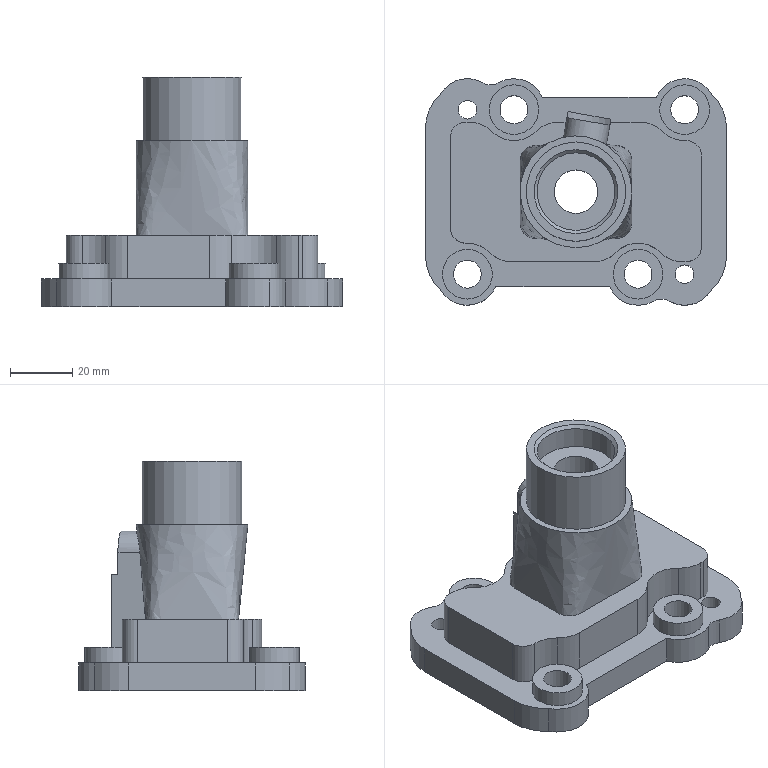Component | NX | CONTROL_COVER | 1 solid | 90 faces | volume 75578 mm3 | cylinder 56 | plane 31 | spline 2 | cone 1 | commonest cylinder face diameters 20 x17 10 x6 23 x6 7 x6 29.479 x4 16 x4 9 x4 14 x2